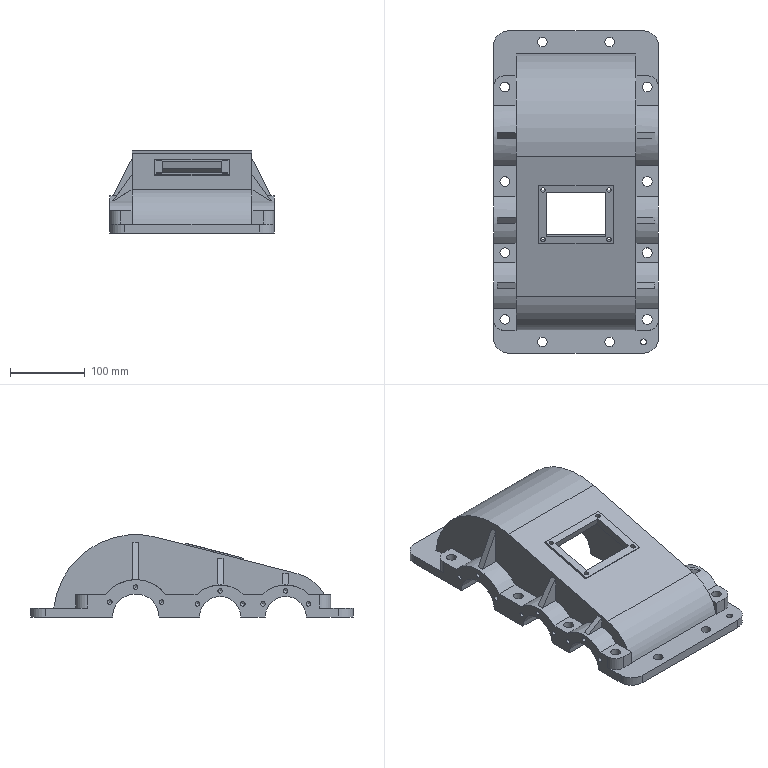Component | NX | XIANGGAI | 1 solid | 136 faces | volume 1574026 mm3 | plane 59 | cylinder 59 | cone 18 | commonest cylinder face diameters 6 x22 13 x12 55 x4 86 x4 30 x4 40 x4 62 x2 100 x2